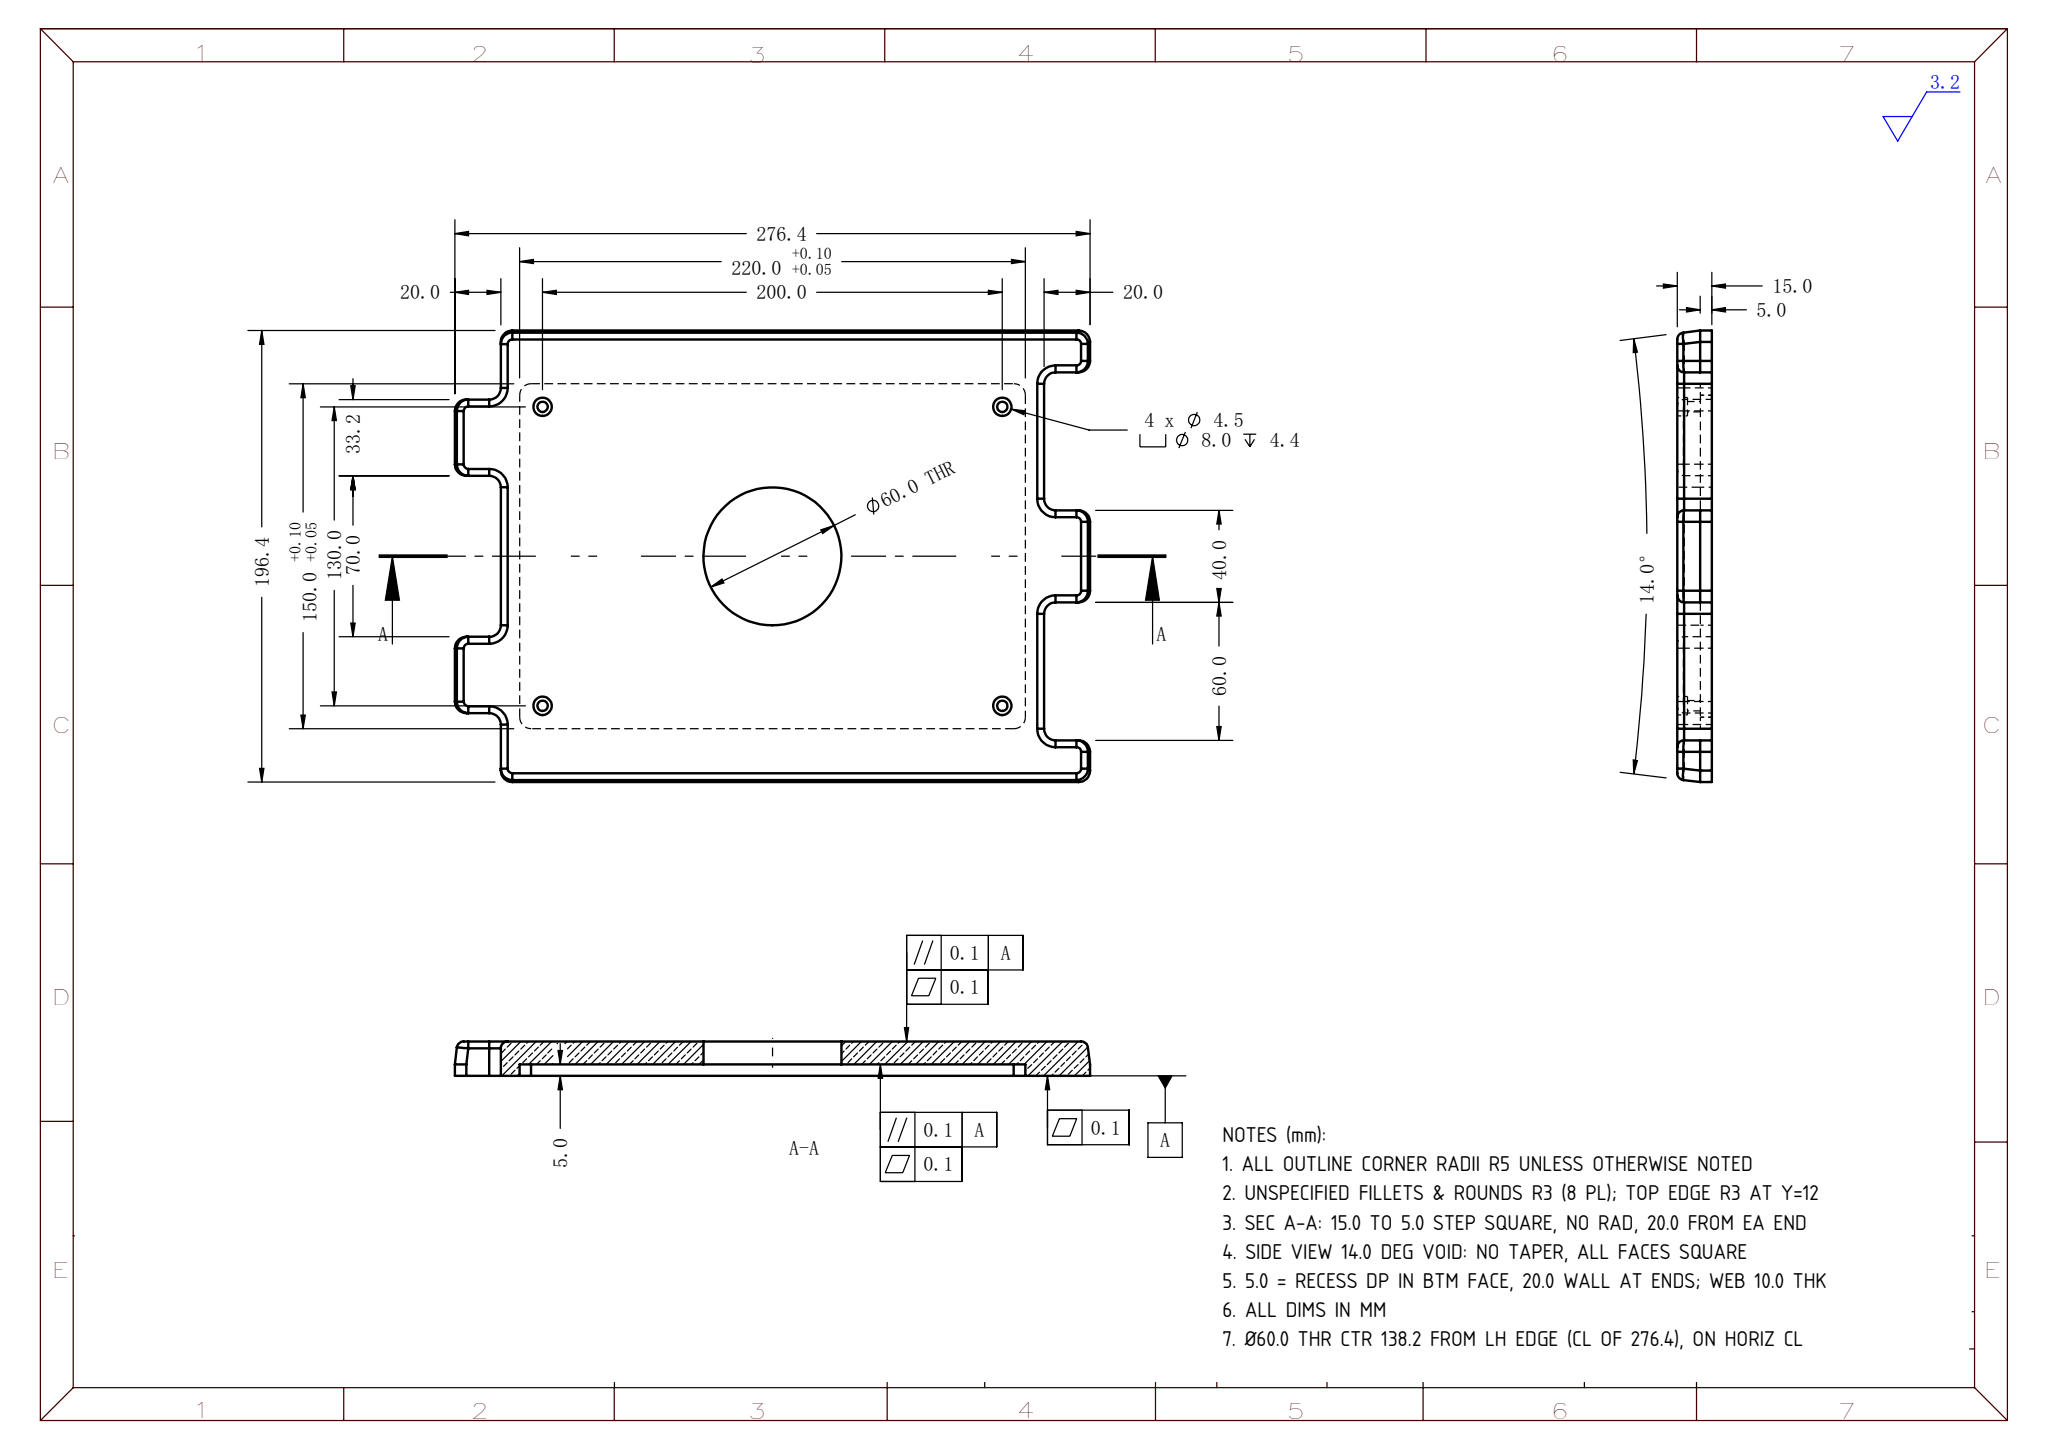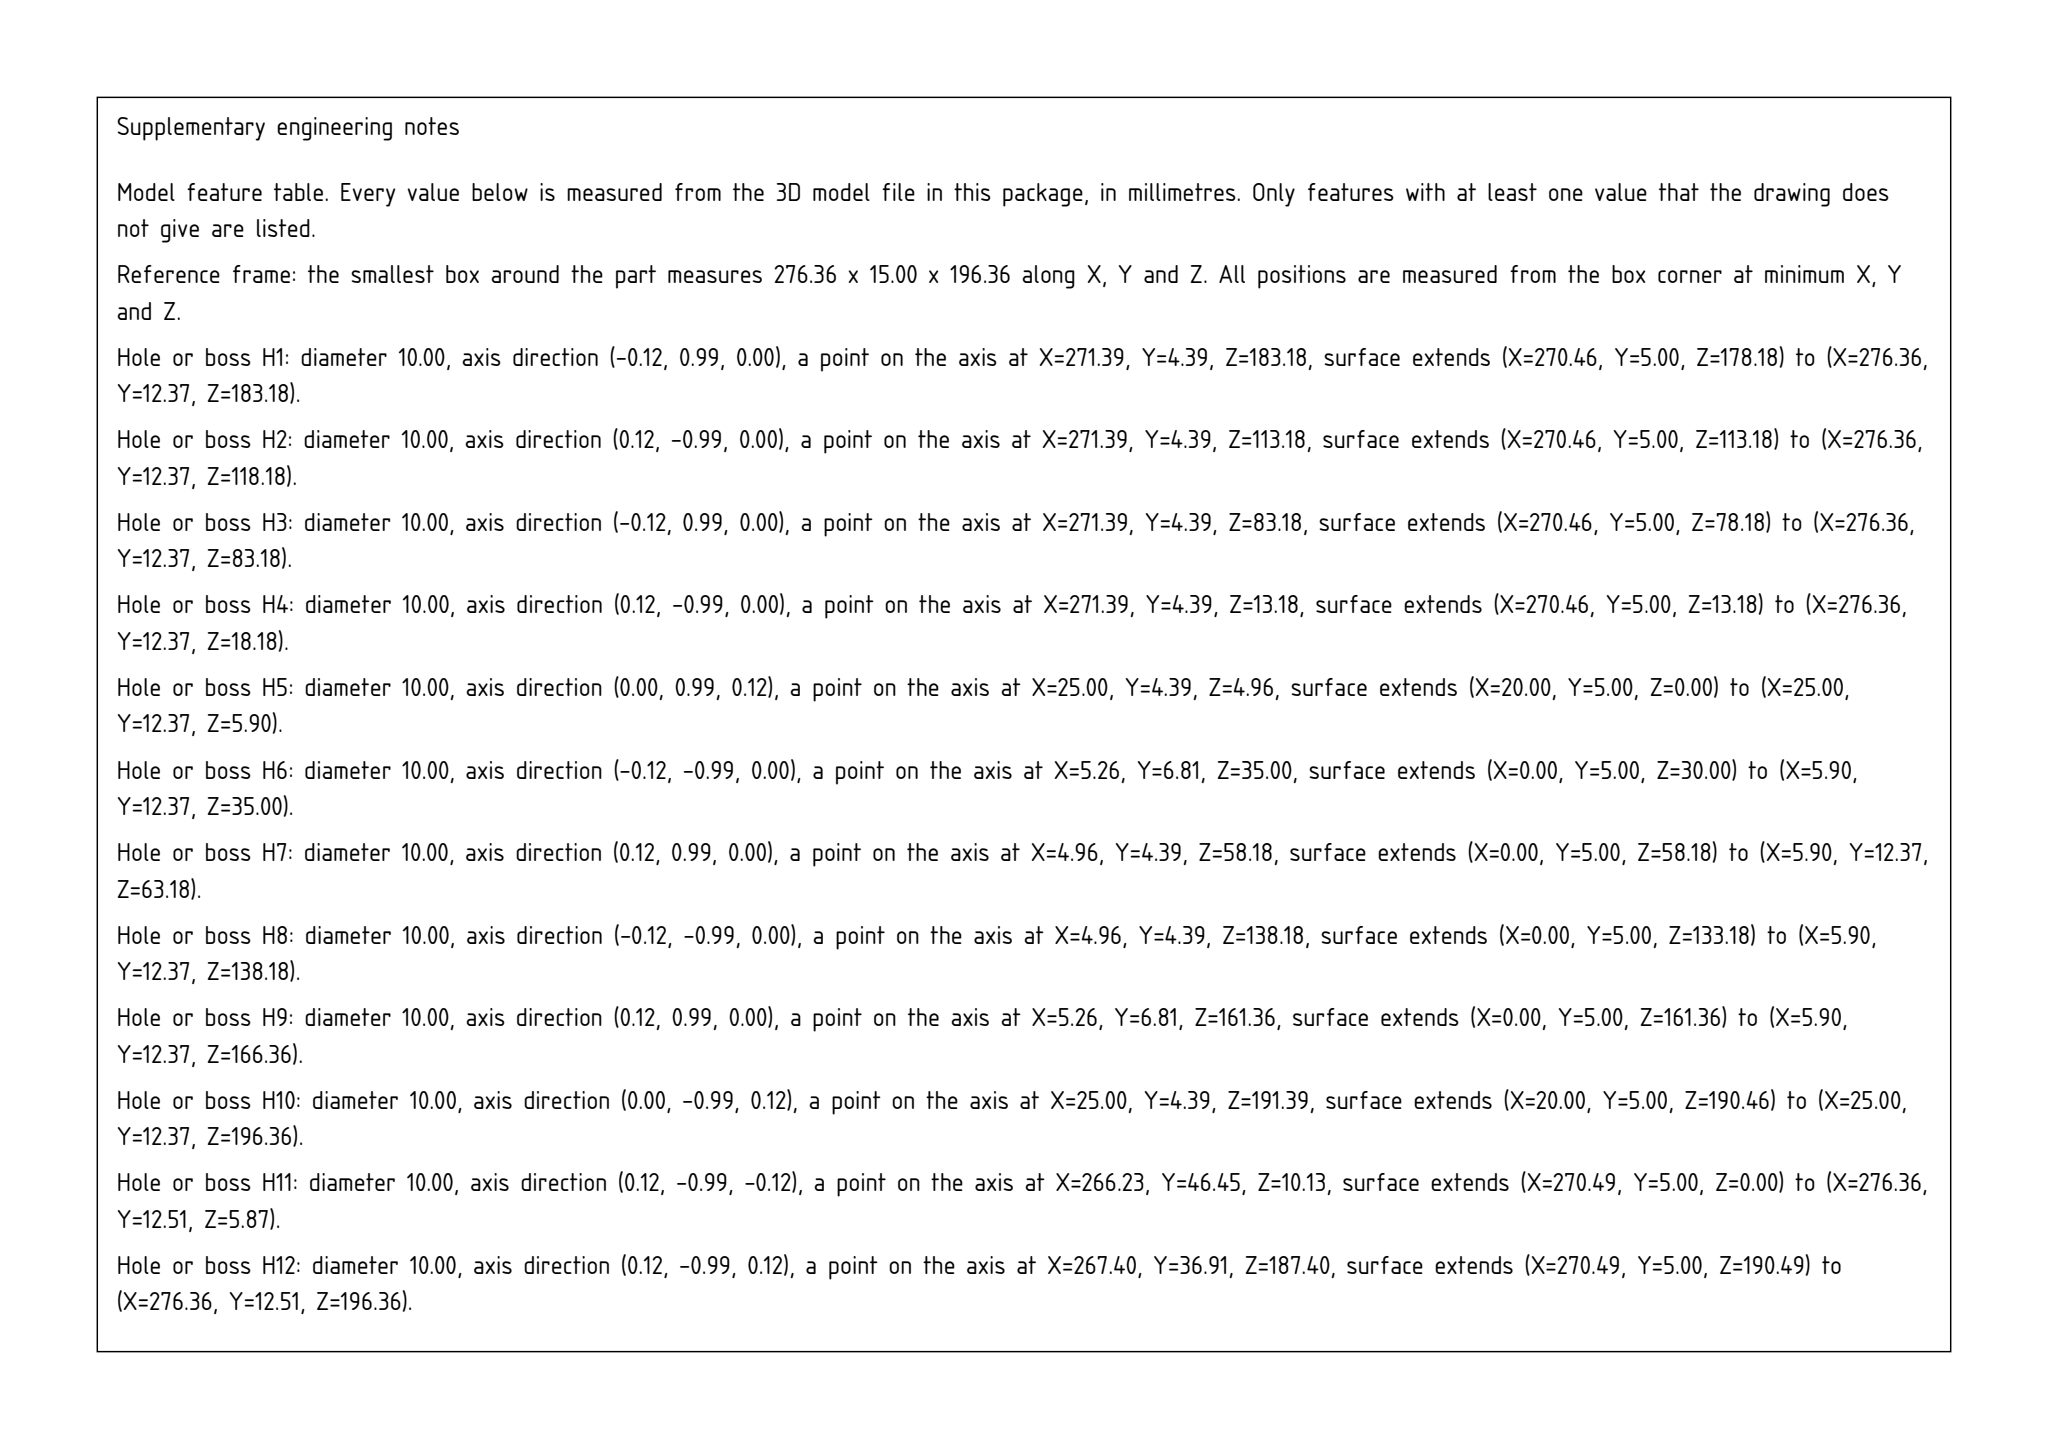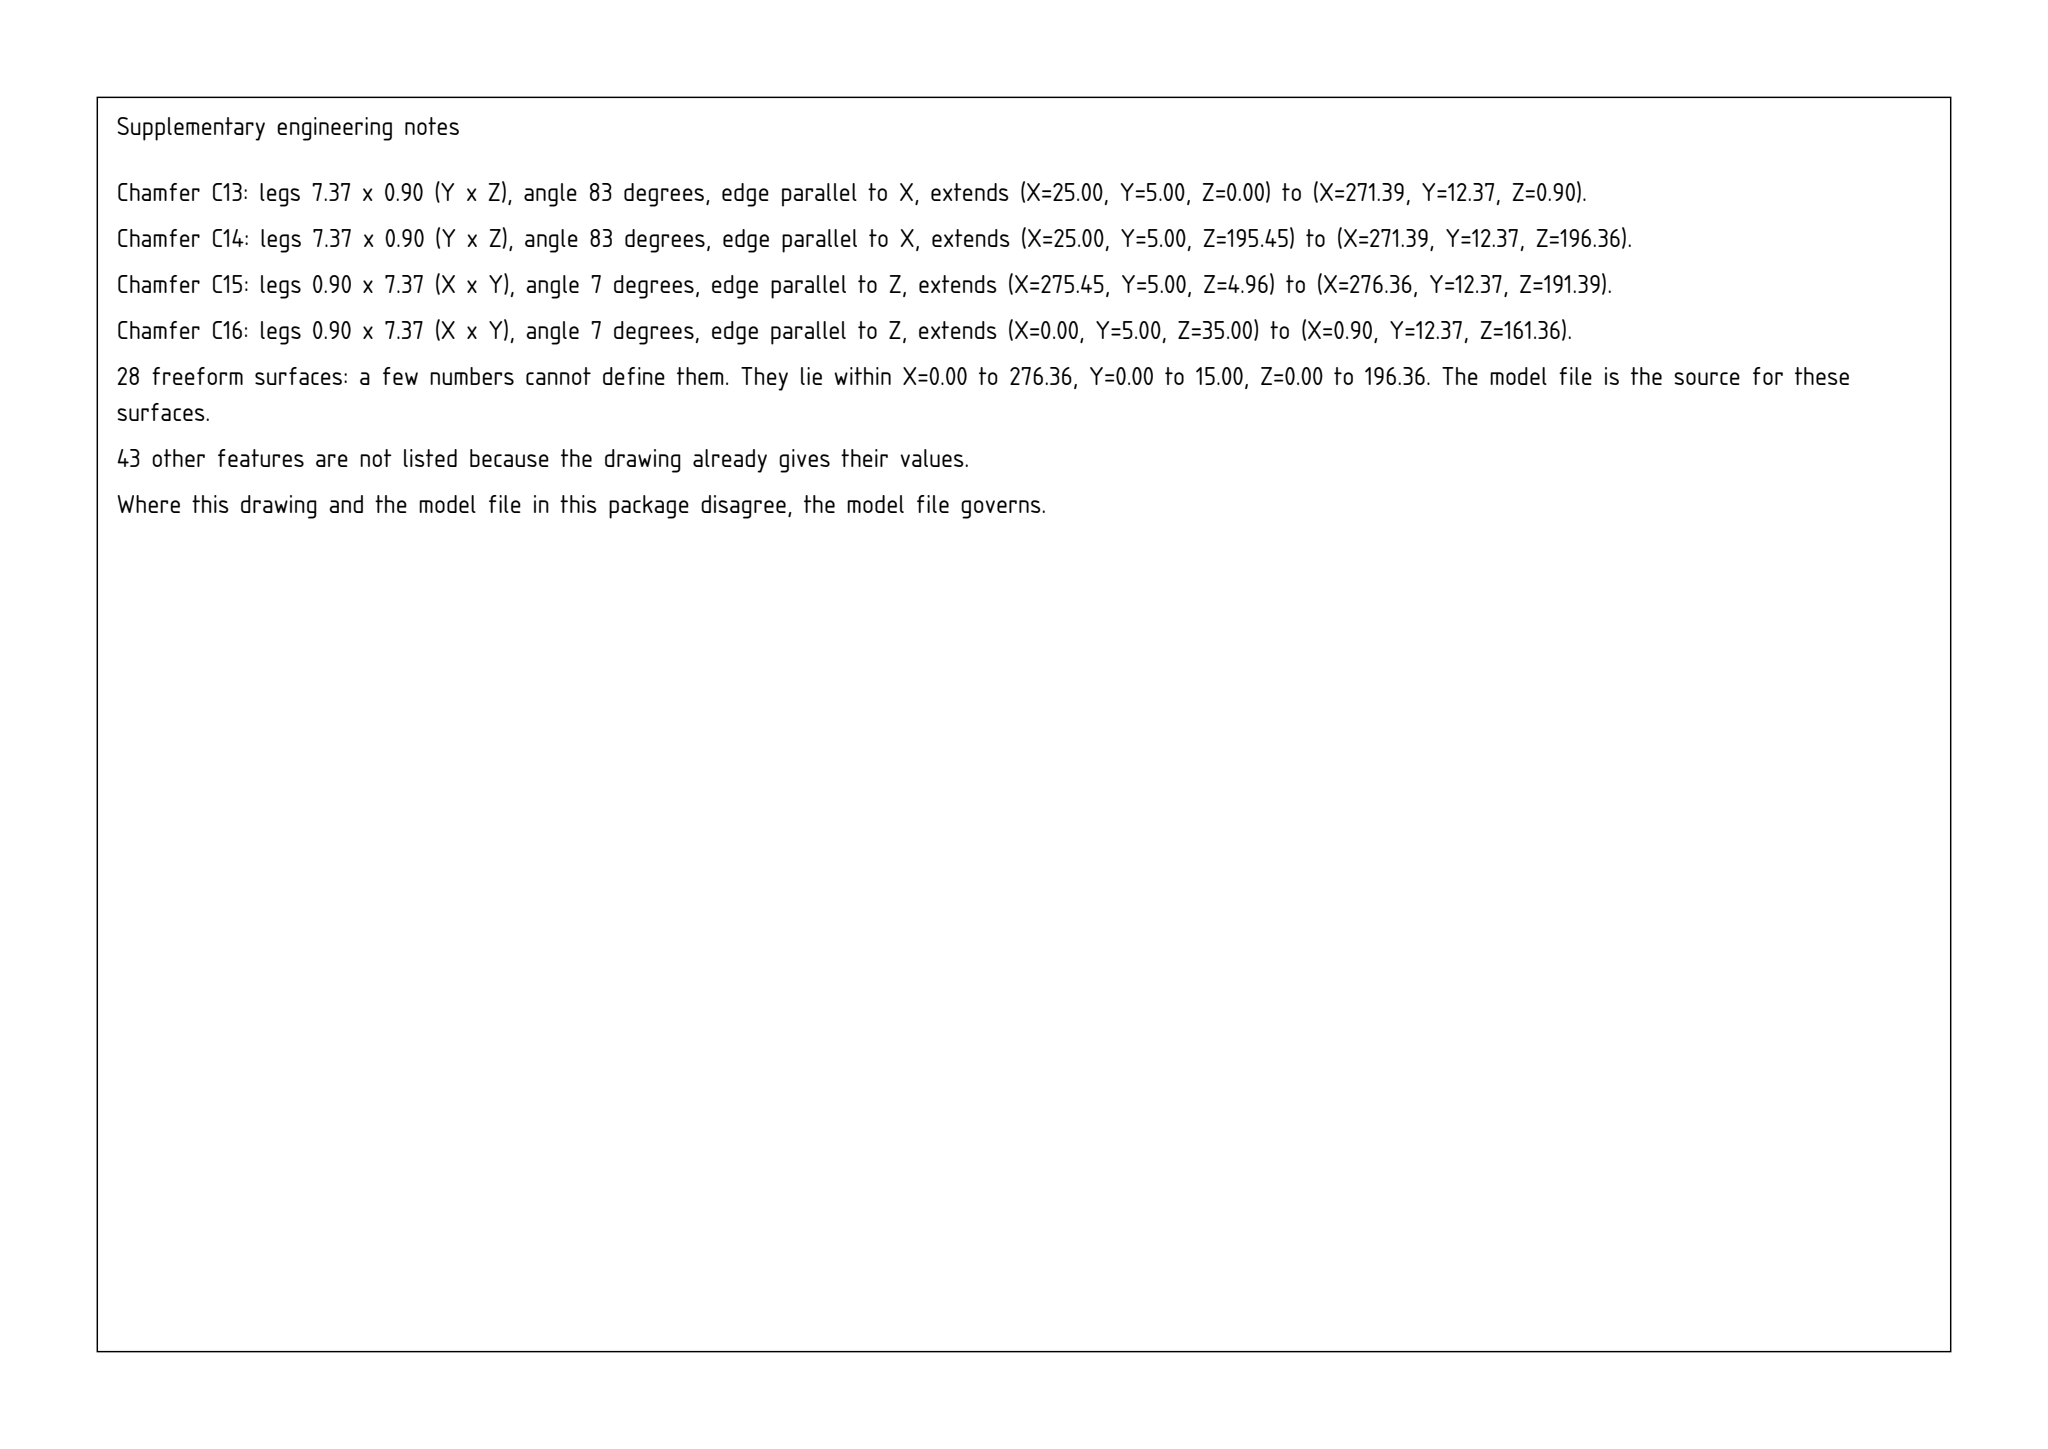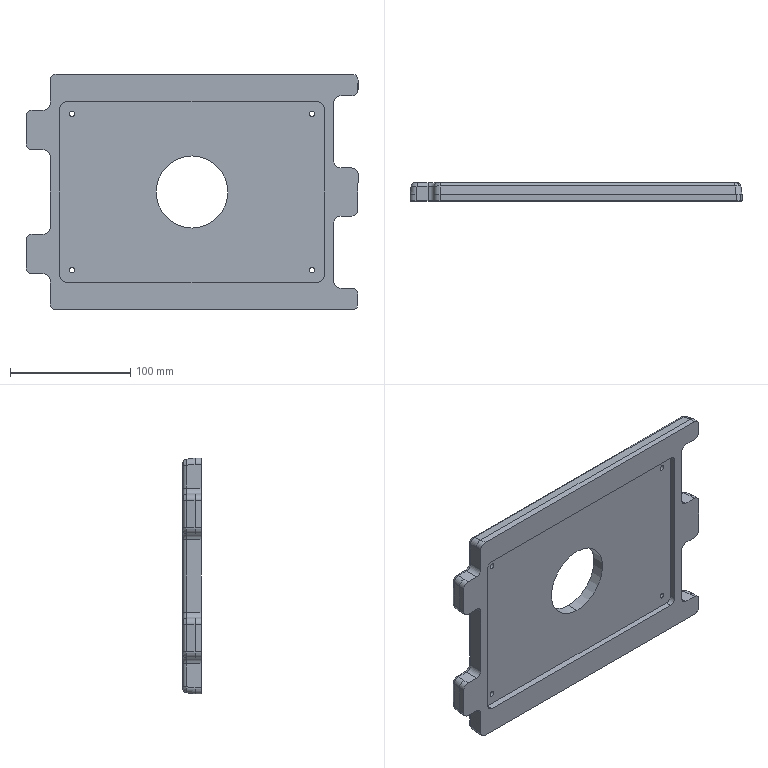Part | SolidWorks | mm | 1 solid | 136 faces | box 276.36 x 15 x 196.36 mm | volume 538589 mm3 | cylinder 62 | plane 38 | spline 28 | torus 8 | commonest cylinder face diameters 10 x24 6 x20 8 x8 4.5 x8 60 x2
Drawing notes:
ALL OUTLINE CORNER RADII R5 UNLESS OTHERWISE NOTED | from the solid: Ø10.0 Y-axis cylinders at all notch/outline corners (R5), e.g. [10.0,'y',[15.0,null,68.21],12.0] and [10.0,'y',[261.36,null,73.21],12.0]
UNSPECIFIED FILLETS & ROUNDS R3 (8 PL); TOP EDGE R3 AT Y=12 | from the solid: fillet_radii [[3.0,8]]; Ø6.0 cylinders on X and Z axes all at y=12.0 (R3 rounded top perimeter edges), e.g. [6.0,'x',[null,12.0,3.91],245.49]
SEC A-A: 15.0 TO 5.0 STEP SQUARE, NO RAD, 20.0 FROM EA END | from the solid: x-normal planes at 20.0 and 256.36 (276.36-256.36=20.0); y planes 0.0/5.0/15.0; no fillet other than R3 x8
SIDE VIEW 14.0 DEG VOID: NO TAPER, ALL FACES SQUARE | from the solid: cones[] empty; all planes axis-normal (x 0/20/28.18/248.18/256.36/276.36, y 0/5/10.6/15, z 0.03...196.39)
5.0 = RECESS DP IN BTM FACE, 20.0 WALL AT ENDS; WEB 10.0 THK | from the solid: y planes 0.0 and 5.0 (single faces) with 15.0 top; Ø60 thru cyl length 10.0; Ø4.5 holes length 5.6 + Ø8.0 c'bore 4.4 = 10.0 web
ALL DIMS IN MM | from the solid: STEP model units mm; bbox_xyz [276.386,15.0,196.416]
Ø60.0 THR CTR 138.2 FROM LH EDGE (CL OF 276.4), ON HORIZ CL | from the solid: cyl dia 60.0 axis y at pos [138.18, -, 98.21]; bbox X=276.386, Z=196.416